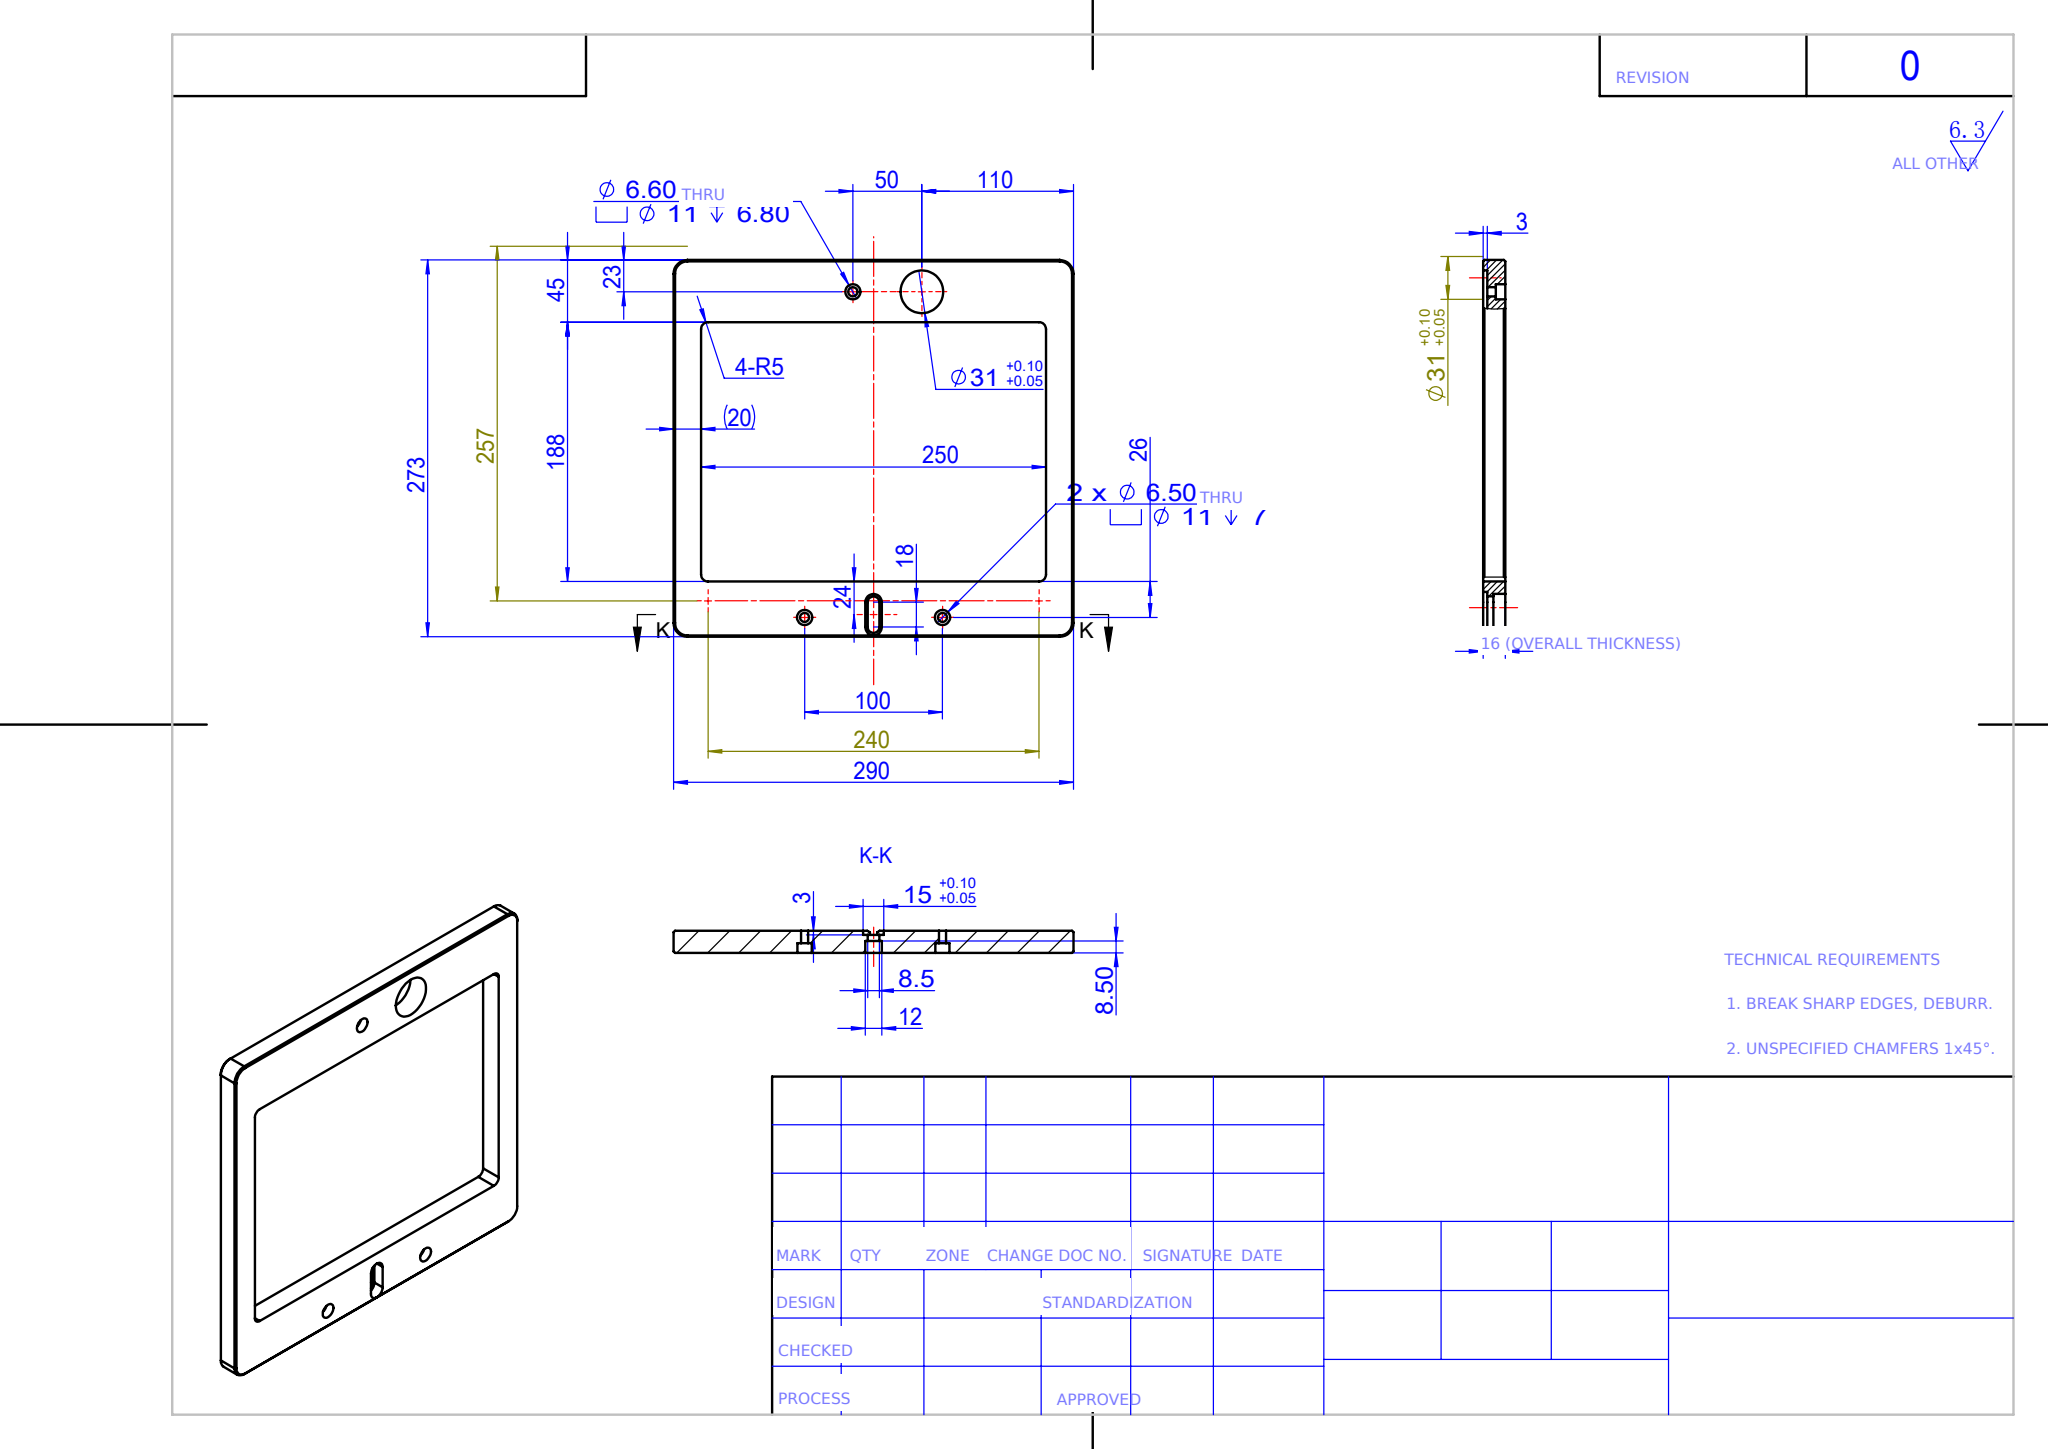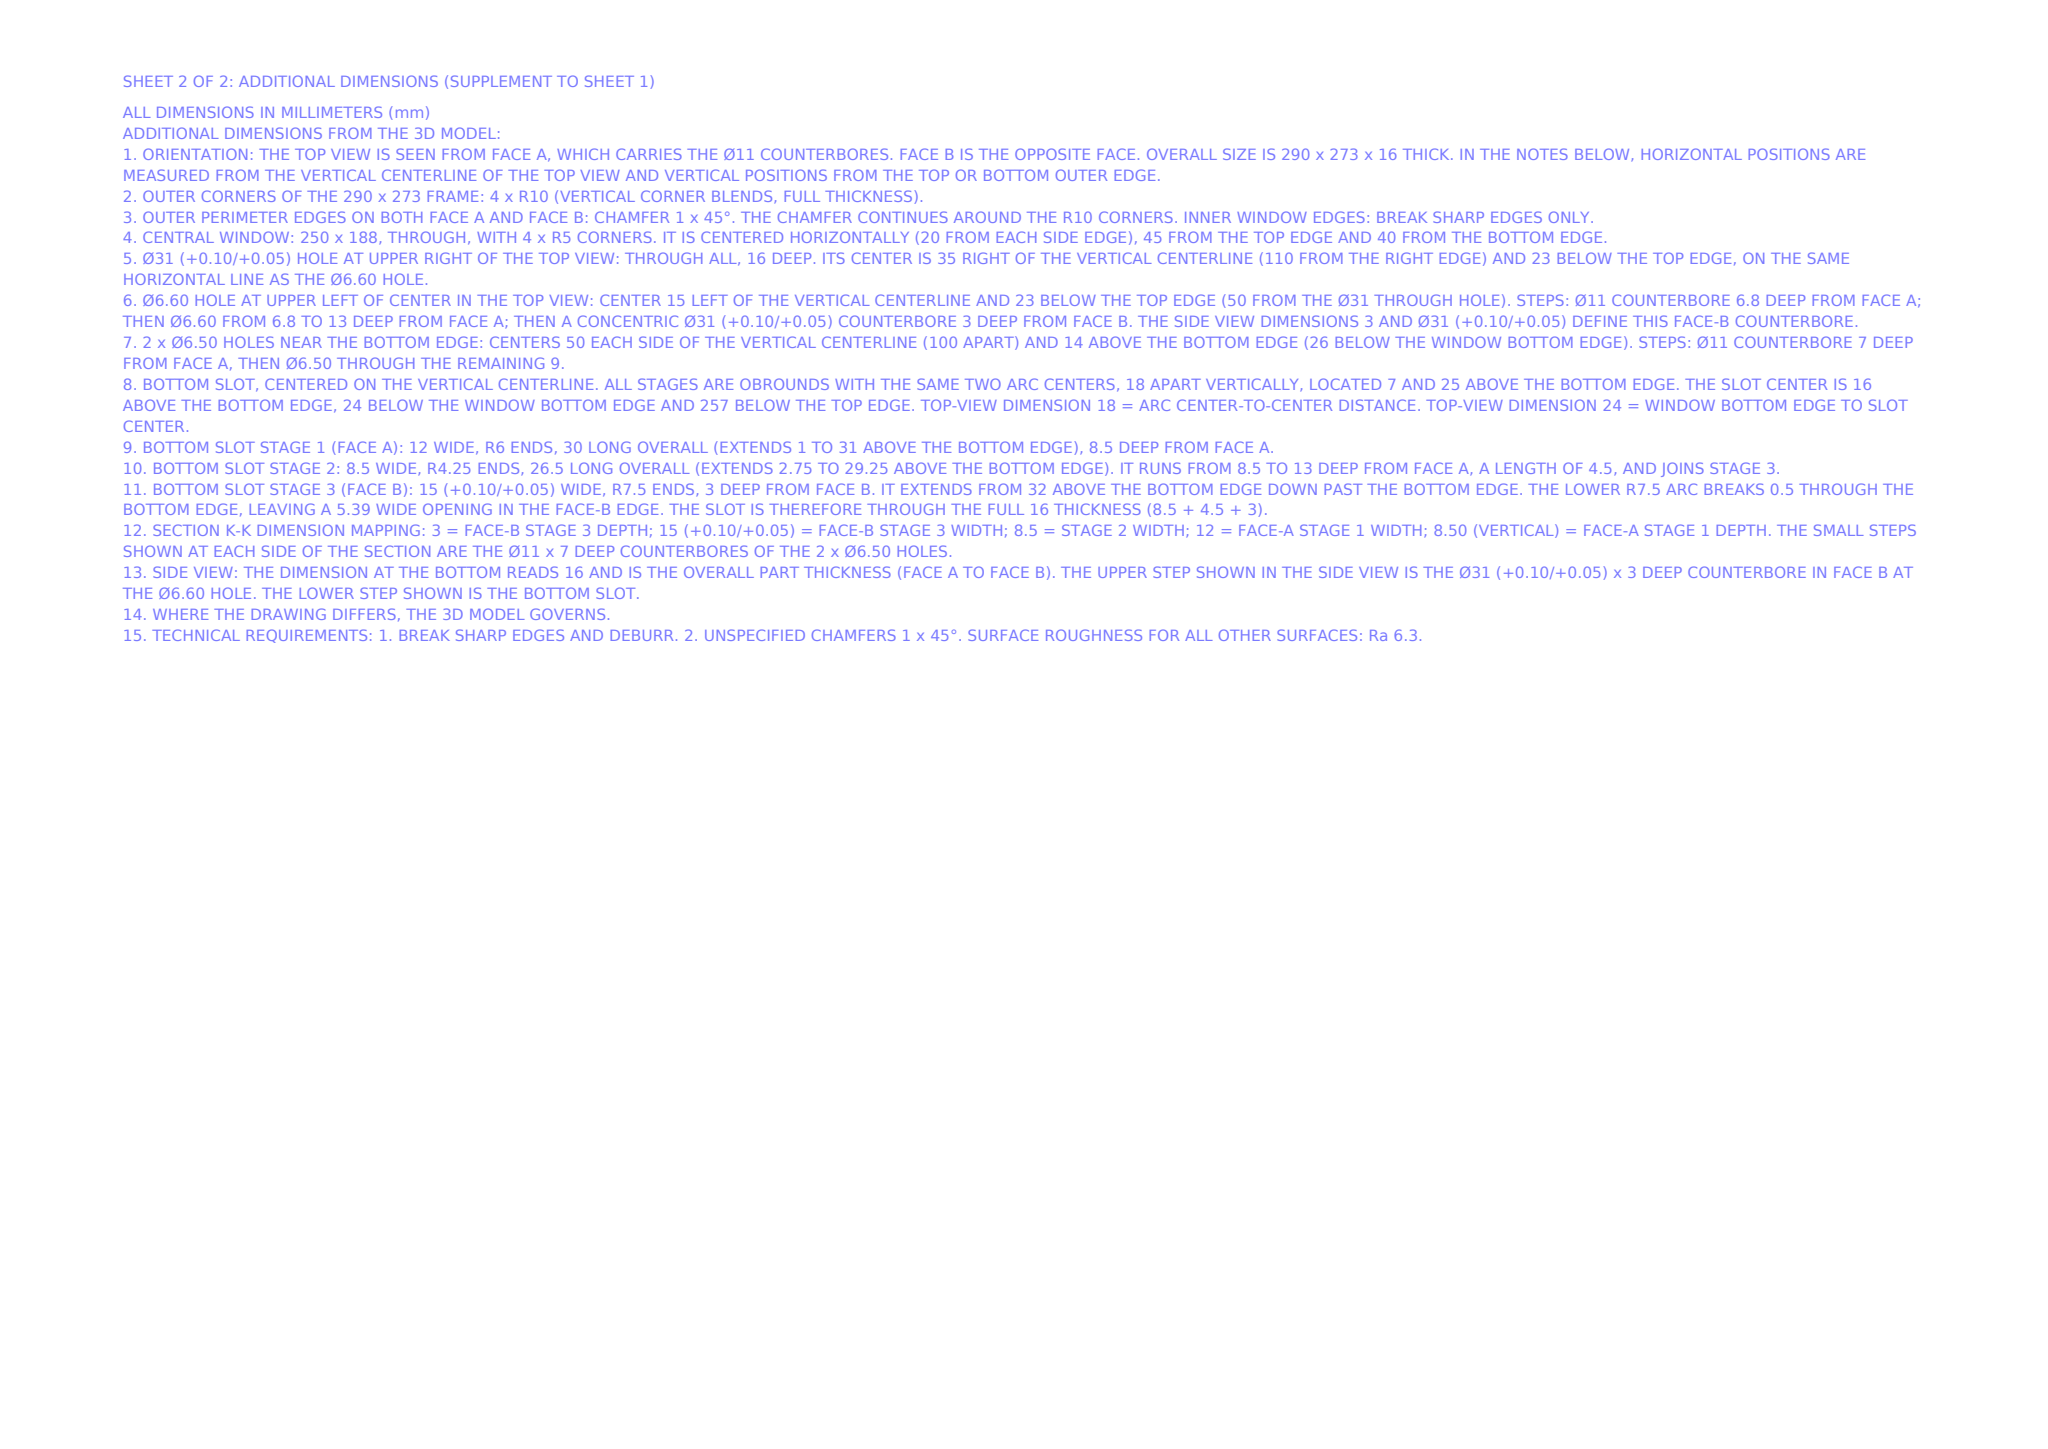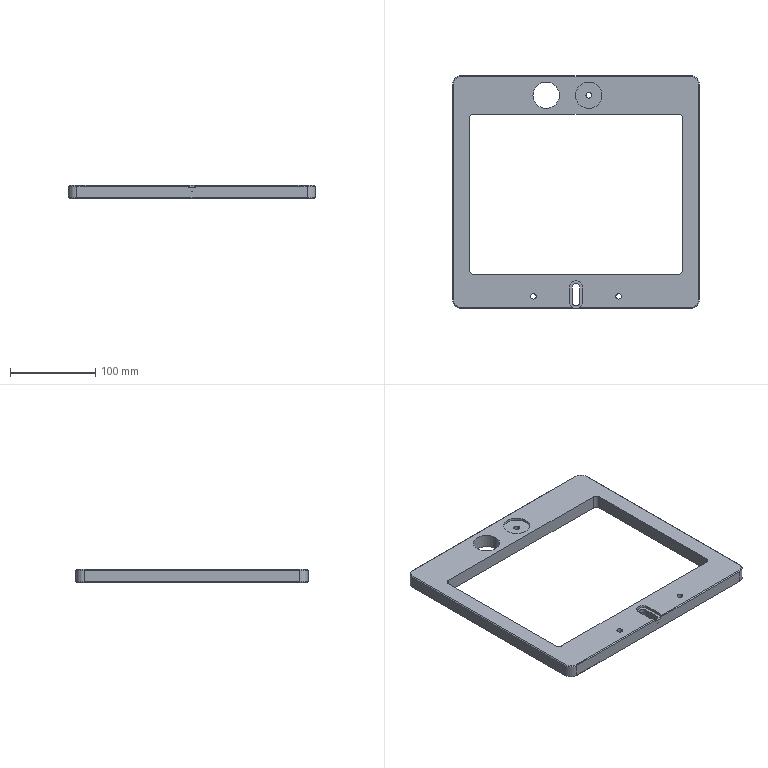Part | NX | mm | 1 solid | 70 faces | box 290 x 273 x 16 mm | volume 490384 mm3 | cylinder 31 | plane 31 | cone 8 | commonest cylinder face diameters 11 x6 6.5 x4 31 x4 10 x4 20 x4 15 x3 6.6 x2 8.5 x2